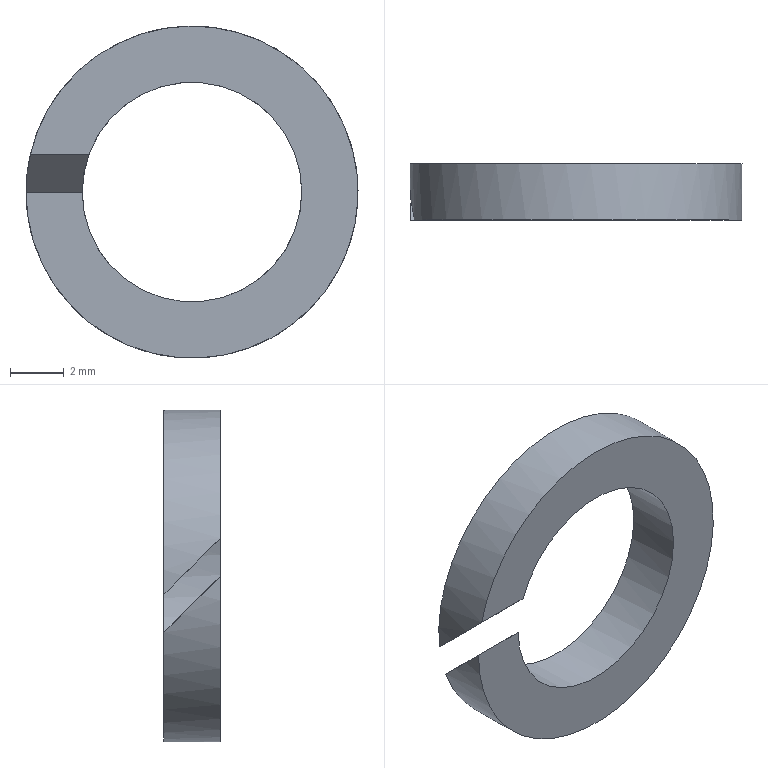Component | NX | SPRING_WASHER_8_3 | 1 solid | 6 faces | box 12.4 x 2.1 x 12.4 mm | volume 136 mm3 | plane 4 | cylinder 2 | commonest cylinder face diameters 12.4 x1 8.2 x1
STEP:
#1=CARTESIAN_POINT('',(0.,0.,0.));
#2=DIRECTION('',(0.,0.,1.));
#3=DIRECTION('',(1.,0.,0.));
#4=AXIS2_PLACEMENT_3D('',#1,#2,#3);
#5=CARTESIAN_POINT('',(-5.834,-94.,-137.1));
#6=VERTEX_POINT('',#5);
#7=CARTESIAN_POINT('',(-6.162,-94.,-135.686));
#8=VERTEX_POINT('',#7);
#9=CARTESIAN_POINT('',(-0.,-94.,-135.));
#10=DIRECTION('',(0.,-1.,0.));
#11=DIRECTION('',(-1.,0.,0.));
#12=AXIS2_PLACEMENT_3D('',#9,#10,#11);
#13=CIRCLE('',#12,6.2);
#14=CARTESIAN_POINT('',(-0.,-94.,-135.));
#15=DIRECTION('',(0.,-1.,0.));
#16=DIRECTION('',(-1.,0.,0.));
#17=AXIS2_PLACEMENT_3D('',#14,#15,#16);
#18=CYLINDRICAL_SURFACE('',#17,6.2);
#19=CARTESIAN_POINT('',(-0.,0.));
#20=DIRECTION('',(1.,0.));
#21=VECTOR('',#20,1.);
#22=LINE('',#19,#21);
#23=(GEOMETRIC_REPRESENTATION_CONTEXT(2)PARAMETRIC_REPRESENTATION_CONTEXT()REPRESENTATION_CONTEXT('',''));
#24=DEFINITIONAL_REPRESENTATION('',(#22),#23);
#25=PCURVE('',#18,#24);
#26=CARTESIAN_POINT('',(-0.,-94.,-135.));
#27=DIRECTION('',(0.,-1.,0.));
#28=DIRECTION('',(-1.,0.,0.));
#29=AXIS2_PLACEMENT_3D('',#26,#27,#28);
#30=PLANE('',#29);
#31=CARTESIAN_POINT('',(0.,0.));
#32=DIRECTION('',(1.,0.));
#33=AXIS2_PLACEMENT_2D('',#31,#32);
#34=CIRCLE('',#33,6.2);
#35=(GEOMETRIC_REPRESENTATION_CONTEXT(2)PARAMETRIC_REPRESENTATION_CONTEXT()REPRESENTATION_CONTEXT('',''));
#36=DEFINITIONAL_REPRESENTATION('',(#34),#35);
#37=PCURVE('',#30,#36);
#38=SURFACE_CURVE('',#13,(#25,#37),.PCURVE_S1.);
#39=EDGE_CURVE('',#6,#8,#38,.T.);
#40=ORIENTED_EDGE('',*,*,#39,.T.);
#41=CARTESIAN_POINT('',(-6.037,-96.1,-133.586));
#42=VERTEX_POINT('',#41);
#43=CARTESIAN_POINT('',(-0.,-94.686,-135.));
#44=DIRECTION('',(0.,0.7071,0.7071));
#45=DIRECTION('',(0.,-0.7071,0.7071));
#46=AXIS2_PLACEMENT_3D('',#43,#44,#45);
#47=ELLIPSE('',#46,8.768,6.2);
#48=CARTESIAN_POINT('',(6.394,-0.));
#49=CARTESIAN_POINT('',(6.053,2.1));
#50=B_SPLINE_CURVE_WITH_KNOTS('',1,(#48,#49),.UNSPECIFIED.,.F.,.F.,(2,2),(4.602,4.943),.PIECEWISE_BEZIER_KNOTS.);
#51=(GEOMETRIC_REPRESENTATION_CONTEXT(2)PARAMETRIC_REPRESENTATION_CONTEXT()REPRESENTATION_CONTEXT('',''));
#52=DEFINITIONAL_REPRESENTATION('',(#50),#51);
#53=PCURVE('',#18,#52);
#54=CARTESIAN_POINT('',(-9.3,-96.528,-133.158));
#55=DIRECTION('',(0.,-0.7071,-0.7071));
#56=DIRECTION('',(0.,-0.7071,0.7071));
#57=AXIS2_PLACEMENT_3D('',#54,#55,#56);
#58=PLANE('',#57);
#59=CARTESIAN_POINT('',(6.164,-9.3));
#60=CARTESIAN_POINT('',(6.164,-20.039));
#61=CARTESIAN_POINT('',(-6.989,-14.669));
#62=CARTESIAN_POINT('',(-20.141,-9.3));
#63=CARTESIAN_POINT('',(-6.989,-3.931));
#64=CARTESIAN_POINT('',(6.164,1.439));
#65=CARTESIAN_POINT('',(6.164,-9.3));
#66=(BOUNDED_CURVE()B_SPLINE_CURVE(2,(#59,#60,#61,#62,#63,#64,#65),.UNSPECIFIED.,.T.,.F.)B_SPLINE_CURVE_WITH_KNOTS((1,2,2,2,2,1),(-2.094,0.,2.094,4.189,6.283,8.378),.UNSPECIFIED.)CURVE()GEOMETRIC_REPRESENTATION_ITEM()RATIONAL_B_SPLINE_CURVE((1.,0.5,1.,0.5,1.,0.5,1.))REPRESENTATION_ITEM(''));
#67=(GEOMETRIC_REPRESENTATION_CONTEXT(2)PARAMETRIC_REPRESENTATION_CONTEXT()REPRESENTATION_CONTEXT('',''));
#68=DEFINITIONAL_REPRESENTATION('',(#66),#67);
#69=PCURVE('',#58,#68);
#70=SURFACE_CURVE('',#47,(#53,#69),.PCURVE_S1.);
#71=EDGE_CURVE('',#8,#42,#70,.T.);
#72=ORIENTED_EDGE('',*,*,#71,.T.);
#73=CARTESIAN_POINT('',(-6.2,-96.1,-135.));
#74=VERTEX_POINT('',#73);
#75=CARTESIAN_POINT('',(-0.,-96.1,-135.));
#76=DIRECTION('',(0.,-1.,0.));
#77=DIRECTION('',(-1.,0.,0.));
#78=AXIS2_PLACEMENT_3D('',#75,#76,#77);
#79=CIRCLE('',#78,6.2);
#80=CARTESIAN_POINT('',(0.,2.1));
#81=DIRECTION('',(1.,0.));
#82=VECTOR('',#81,1.);
#83=LINE('',#80,#82);
#84=(GEOMETRIC_REPRESENTATION_CONTEXT(2)PARAMETRIC_REPRESENTATION_CONTEXT()REPRESENTATION_CONTEXT('',''));
#85=DEFINITIONAL_REPRESENTATION('',(#83),#84);
#86=PCURVE('',#18,#85);
#87=CARTESIAN_POINT('',(-0.,-96.1,-135.));
#88=DIRECTION('',(0.,-1.,0.));
#89=DIRECTION('',(-1.,0.,0.));
#90=AXIS2_PLACEMENT_3D('',#87,#88,#89);
#91=PLANE('',#90);
#92=CARTESIAN_POINT('',(0.,0.));
#93=DIRECTION('',(1.,0.));
#94=AXIS2_PLACEMENT_2D('',#92,#93);
#95=CIRCLE('',#94,6.2);
#96=(GEOMETRIC_REPRESENTATION_CONTEXT(2)PARAMETRIC_REPRESENTATION_CONTEXT()REPRESENTATION_CONTEXT('',''));
#97=DEFINITIONAL_REPRESENTATION('',(#95),#96);
#98=PCURVE('',#91,#97);
#99=SURFACE_CURVE('',#79,(#86,#98),.PCURVE_S1.);
#100=EDGE_CURVE('',#74,#42,#99,.T.);
#101=ORIENTED_EDGE('',*,*,#100,.F.);
#102=CARTESIAN_POINT('',(-0.,-96.1,-135.));
#103=DIRECTION('',(0.,-0.7071,-0.7071));
#104=DIRECTION('',(0.,-0.7071,0.7071));
#105=AXIS2_PLACEMENT_3D('',#102,#103,#104);
#106=ELLIPSE('',#105,8.768,6.2);
#107=CARTESIAN_POINT('',(0.,2.1));
#108=CARTESIAN_POINT('',(0.3455,0.));
#109=B_SPLINE_CURVE_WITH_KNOTS('',1,(#107,#108),.UNSPECIFIED.,.F.,.F.,(2,2),(1.571,1.916),.PIECEWISE_BEZIER_KNOTS.);
#110=(GEOMETRIC_REPRESENTATION_CONTEXT(2)PARAMETRIC_REPRESENTATION_CONTEXT()REPRESENTATION_CONTEXT('',''));
#111=DEFINITIONAL_REPRESENTATION('',(#109),#110);
#112=PCURVE('',#18,#111);
#113=CARTESIAN_POINT('',(-9.3,-93.317,-137.783));
#114=DIRECTION('',(0.,0.7071,0.7071));
#115=DIRECTION('',(0.,0.7071,-0.7071));
#116=AXIS2_PLACEMENT_3D('',#113,#114,#115);
#117=PLANE('',#116);
#118=CARTESIAN_POINT('',(-12.704,-9.3));
#119=CARTESIAN_POINT('',(-12.704,1.439));
#120=CARTESIAN_POINT('',(0.4481,-3.931));
#121=CARTESIAN_POINT('',(13.6,-9.3));
#122=CARTESIAN_POINT('',(0.4481,-14.669));
#123=CARTESIAN_POINT('',(-12.704,-20.039));
#124=CARTESIAN_POINT('',(-12.704,-9.3));
#125=(BOUNDED_CURVE()B_SPLINE_CURVE(2,(#118,#119,#120,#121,#122,#123,#124),.UNSPECIFIED.,.T.,.F.)B_SPLINE_CURVE_WITH_KNOTS((1,2,2,2,2,1),(-2.094,0.,2.094,4.189,6.283,8.378),.UNSPECIFIED.)CURVE()GEOMETRIC_REPRESENTATION_ITEM()RATIONAL_B_SPLINE_CURVE((1.,0.5,1.,0.5,1.,0.5,1.))REPRESENTATION_ITEM(''));
#126=(GEOMETRIC_REPRESENTATION_CONTEXT(2)PARAMETRIC_REPRESENTATION_CONTEXT()REPRESENTATION_CONTEXT('',''));
#127=DEFINITIONAL_REPRESENTATION('',(#125),#126);
#128=PCURVE('',#117,#127);
#129=SURFACE_CURVE('',#106,(#112,#128),.PCURVE_S1.);
#130=EDGE_CURVE('',#74,#6,#129,.T.);
#131=ORIENTED_EDGE('',*,*,#130,.T.);
#132=EDGE_LOOP('',(#40,#72,#101,#131));
#133=FACE_BOUND('',#132,.T.);
#134=ADVANCED_FACE('',(#133),#18,.T.);
#135=CARTESIAN_POINT('',(-4.1,-96.1,-135.));
#136=VERTEX_POINT('',#135);
#137=CARTESIAN_POINT('',(-3.848,-96.1,-133.586));
#138=VERTEX_POINT('',#137);
#139=CARTESIAN_POINT('',(-0.,-96.1,-135.));
#140=DIRECTION('',(0.,-1.,0.));
#141=DIRECTION('',(-1.,0.,0.));
#142=AXIS2_PLACEMENT_3D('',#139,#140,#141);
#143=CIRCLE('',#142,4.1);
#144=CARTESIAN_POINT('',(-0.,-94.,-135.));
#145=DIRECTION('',(0.,-1.,0.));
#146=DIRECTION('',(-1.,0.,0.));
#147=AXIS2_PLACEMENT_3D('',#144,#145,#146);
#148=CYLINDRICAL_SURFACE('',#147,4.1);
#149=CARTESIAN_POINT('',(0.,2.1));
#150=DIRECTION('',(1.,0.));
#151=VECTOR('',#150,1.);
#152=LINE('',#149,#151);
#153=(GEOMETRIC_REPRESENTATION_CONTEXT(2)PARAMETRIC_REPRESENTATION_CONTEXT()REPRESENTATION_CONTEXT('',''));
#154=DEFINITIONAL_REPRESENTATION('',(#152),#153);
#155=PCURVE('',#148,#154);
#156=CARTESIAN_POINT('',(0.,0.));
#157=DIRECTION('',(1.,0.));
#158=AXIS2_PLACEMENT_2D('',#156,#157);
#159=CIRCLE('',#158,4.1);
#160=(GEOMETRIC_REPRESENTATION_CONTEXT(2)PARAMETRIC_REPRESENTATION_CONTEXT()REPRESENTATION_CONTEXT('',''));
#161=DEFINITIONAL_REPRESENTATION('',(#159),#160);
#162=PCURVE('',#91,#161);
#163=SURFACE_CURVE('',#143,(#155,#162),.PCURVE_S1.);
#164=EDGE_CURVE('',#136,#138,#163,.T.);
#165=ORIENTED_EDGE('',*,*,#164,.F.);
#166=CARTESIAN_POINT('',(-3.521,-94.,-137.1));
#167=VERTEX_POINT('',#166);
#168=CARTESIAN_POINT('',(-0.,-96.1,-135.));
#169=DIRECTION('',(0.,-0.7071,-0.7071));
#170=DIRECTION('',(0.,-0.7071,0.7071));
#171=AXIS2_PLACEMENT_3D('',#168,#169,#170);
#172=ELLIPSE('',#171,5.798,4.1);
#173=CARTESIAN_POINT('',(0.,2.1));
#174=CARTESIAN_POINT('',(0.5377,0.));
#175=B_SPLINE_CURVE_WITH_KNOTS('',1,(#173,#174),.UNSPECIFIED.,.F.,.F.,(2,2),(1.571,2.109),.PIECEWISE_BEZIER_KNOTS.);
#176=(GEOMETRIC_REPRESENTATION_CONTEXT(2)PARAMETRIC_REPRESENTATION_CONTEXT()REPRESENTATION_CONTEXT('',''));
#177=DEFINITIONAL_REPRESENTATION('',(#175),#176);
#178=PCURVE('',#148,#177);
#179=CARTESIAN_POINT('',(-9.734,-9.3));
#180=CARTESIAN_POINT('',(-9.734,-2.199));
#181=CARTESIAN_POINT('',(-1.037,-5.749));
#182=CARTESIAN_POINT('',(7.661,-9.3));
#183=CARTESIAN_POINT('',(-1.037,-12.851));
#184=CARTESIAN_POINT('',(-9.734,-16.401));
#185=CARTESIAN_POINT('',(-9.734,-9.3));
#186=(BOUNDED_CURVE()B_SPLINE_CURVE(2,(#179,#180,#181,#182,#183,#184,#185),.UNSPECIFIED.,.T.,.F.)B_SPLINE_CURVE_WITH_KNOTS((1,2,2,2,2,1),(-2.094,0.,2.094,4.189,6.283,8.378),.UNSPECIFIED.)CURVE()GEOMETRIC_REPRESENTATION_ITEM()RATIONAL_B_SPLINE_CURVE((1.,0.5,1.,0.5,1.,0.5,1.))REPRESENTATION_ITEM(''));
#187=(GEOMETRIC_REPRESENTATION_CONTEXT(2)PARAMETRIC_REPRESENTATION_CONTEXT()REPRESENTATION_CONTEXT('',''));
#188=DEFINITIONAL_REPRESENTATION('',(#186),#187);
#189=PCURVE('',#117,#188);
#190=SURFACE_CURVE('',#172,(#178,#189),.PCURVE_S1.);
#191=EDGE_CURVE('',#136,#167,#190,.T.);
#192=ORIENTED_EDGE('',*,*,#191,.T.);
#193=CARTESIAN_POINT('',(-4.042,-94.,-135.686));
#194=VERTEX_POINT('',#193);
#195=CARTESIAN_POINT('',(-0.,-94.,-135.));
#196=DIRECTION('',(0.,-1.,0.));
#197=DIRECTION('',(-1.,0.,0.));
#198=AXIS2_PLACEMENT_3D('',#195,#196,#197);
#199=CIRCLE('',#198,4.1);
#200=CARTESIAN_POINT('',(-0.,0.));
#201=DIRECTION('',(1.,0.));
#202=VECTOR('',#201,1.);
#203=LINE('',#200,#202);
#204=(GEOMETRIC_REPRESENTATION_CONTEXT(2)PARAMETRIC_REPRESENTATION_CONTEXT()REPRESENTATION_CONTEXT('',''));
#205=DEFINITIONAL_REPRESENTATION('',(#203),#204);
#206=PCURVE('',#148,#205);
#207=CARTESIAN_POINT('',(0.,0.));
#208=DIRECTION('',(1.,0.));
#209=AXIS2_PLACEMENT_2D('',#207,#208);
#210=CIRCLE('',#209,4.1);
#211=(GEOMETRIC_REPRESENTATION_CONTEXT(2)PARAMETRIC_REPRESENTATION_CONTEXT()REPRESENTATION_CONTEXT('',''));
#212=DEFINITIONAL_REPRESENTATION('',(#210),#211);
#213=PCURVE('',#30,#212);
#214=SURFACE_CURVE('',#199,(#206,#213),.PCURVE_S1.);
#215=EDGE_CURVE('',#167,#194,#214,.T.);
#216=ORIENTED_EDGE('',*,*,#215,.T.);
#217=CARTESIAN_POINT('',(-0.,-94.686,-135.));
#218=DIRECTION('',(0.,0.7071,0.7071));
#219=DIRECTION('',(0.,-0.7071,0.7071));
#220=AXIS2_PLACEMENT_3D('',#217,#218,#219);
#221=ELLIPSE('',#220,5.798,4.1);
#222=CARTESIAN_POINT('',(6.451,-0.));
#223=CARTESIAN_POINT('',(5.931,2.1));
#224=B_SPLINE_CURVE_WITH_KNOTS('',1,(#222,#223),.UNSPECIFIED.,.F.,.F.,(2,2),(4.544,5.065),.PIECEWISE_BEZIER_KNOTS.);
#225=(GEOMETRIC_REPRESENTATION_CONTEXT(2)PARAMETRIC_REPRESENTATION_CONTEXT()REPRESENTATION_CONTEXT('',''));
#226=DEFINITIONAL_REPRESENTATION('',(#224),#225);
#227=PCURVE('',#148,#226);
#228=CARTESIAN_POINT('',(3.194,-9.3));
#229=CARTESIAN_POINT('',(3.194,-16.401));
#230=CARTESIAN_POINT('',(-5.504,-12.851));
#231=CARTESIAN_POINT('',(-14.201,-9.3));
#232=CARTESIAN_POINT('',(-5.504,-5.749));
#233=CARTESIAN_POINT('',(3.194,-2.199));
#234=CARTESIAN_POINT('',(3.194,-9.3));
#235=(BOUNDED_CURVE()B_SPLINE_CURVE(2,(#228,#229,#230,#231,#232,#233,#234),.UNSPECIFIED.,.T.,.F.)B_SPLINE_CURVE_WITH_KNOTS((1,2,2,2,2,1),(-2.094,0.,2.094,4.189,6.283,8.378),.UNSPECIFIED.)CURVE()GEOMETRIC_REPRESENTATION_ITEM()RATIONAL_B_SPLINE_CURVE((1.,0.5,1.,0.5,1.,0.5,1.))REPRESENTATION_ITEM(''));
#236=(GEOMETRIC_REPRESENTATION_CONTEXT(2)PARAMETRIC_REPRESENTATION_CONTEXT()REPRESENTATION_CONTEXT('',''));
#237=DEFINITIONAL_REPRESENTATION('',(#235),#236);
#238=PCURVE('',#58,#237);
#239=SURFACE_CURVE('',#221,(#227,#238),.PCURVE_S1.);
#240=EDGE_CURVE('',#194,#138,#239,.T.);
#241=ORIENTED_EDGE('',*,*,#240,.T.);
#242=EDGE_LOOP('',(#165,#192,#216,#241));
#243=FACE_BOUND('',#242,.F.);
#244=ADVANCED_FACE('',(#243),#148,.F.);
#245=CARTESIAN_POINT('',(-0.,-94.,-135.686));
#246=DIRECTION('',(1.,0.,0.));
#247=VECTOR('',#246,1.);
#248=LINE('',#245,#247);
#249=CARTESIAN_POINT('',(0.,0.6858));
#250=DIRECTION('',(-1.,0.));
#251=VECTOR('',#250,1.);
#252=LINE('',#249,#251);
#253=(GEOMETRIC_REPRESENTATION_CONTEXT(2)PARAMETRIC_REPRESENTATION_CONTEXT()REPRESENTATION_CONTEXT('',''));
#254=DEFINITIONAL_REPRESENTATION('',(#252),#253);
#255=PCURVE('',#30,#254);
#256=CARTESIAN_POINT('',(-3.574,-9.3));
#257=DIRECTION('',(0.,-1.));
#258=VECTOR('',#257,1.);
#259=LINE('',#256,#258);
#260=(GEOMETRIC_REPRESENTATION_CONTEXT(2)PARAMETRIC_REPRESENTATION_CONTEXT()REPRESENTATION_CONTEXT('',''));
#261=DEFINITIONAL_REPRESENTATION('',(#259),#260);
#262=PCURVE('',#58,#261);
#263=SURFACE_CURVE('',#248,(#255,#262),.PCURVE_S1.);
#264=EDGE_CURVE('',#8,#194,#263,.T.);
#265=ORIENTED_EDGE('',*,*,#264,.F.);
#266=ORIENTED_EDGE('',*,*,#39,.F.);
#267=CARTESIAN_POINT('',(-0.,-94.,-137.1));
#268=DIRECTION('',(-1.,0.,0.));
#269=VECTOR('',#268,1.);
#270=LINE('',#267,#269);
#271=CARTESIAN_POINT('',(0.,2.1));
#272=DIRECTION('',(1.,0.));
#273=VECTOR('',#272,1.);
#274=LINE('',#271,#273);
#275=(GEOMETRIC_REPRESENTATION_CONTEXT(2)PARAMETRIC_REPRESENTATION_CONTEXT()REPRESENTATION_CONTEXT('',''));
#276=DEFINITIONAL_REPRESENTATION('',(#274),#275);
#277=PCURVE('',#30,#276);
#278=CARTESIAN_POINT('',(-0.9661,-9.3));
#279=DIRECTION('',(0.,1.));
#280=VECTOR('',#279,1.);
#281=LINE('',#278,#280);
#282=(GEOMETRIC_REPRESENTATION_CONTEXT(2)PARAMETRIC_REPRESENTATION_CONTEXT()REPRESENTATION_CONTEXT('',''));
#283=DEFINITIONAL_REPRESENTATION('',(#281),#282);
#284=PCURVE('',#117,#283);
#285=SURFACE_CURVE('',#270,(#277,#284),.PCURVE_S1.);
#286=EDGE_CURVE('',#167,#6,#285,.T.);
#287=ORIENTED_EDGE('',*,*,#286,.F.);
#288=ORIENTED_EDGE('',*,*,#215,.T.);
#289=EDGE_LOOP('',(#265,#266,#287,#288));
#290=FACE_BOUND('',#289,.T.);
#291=ADVANCED_FACE('',(#290),#30,.F.);
#292=ORIENTED_EDGE('',*,*,#100,.T.);
#293=CARTESIAN_POINT('',(-0.,-96.1,-133.586));
#294=DIRECTION('',(1.,0.,0.));
#295=VECTOR('',#294,1.);
#296=LINE('',#293,#295);
#297=CARTESIAN_POINT('',(0.,-1.414));
#298=DIRECTION('',(-1.,0.));
#299=VECTOR('',#298,1.);
#300=LINE('',#297,#299);
#301=(GEOMETRIC_REPRESENTATION_CONTEXT(2)PARAMETRIC_REPRESENTATION_CONTEXT()REPRESENTATION_CONTEXT('',''));
#302=DEFINITIONAL_REPRESENTATION('',(#300),#301);
#303=PCURVE('',#91,#302);
#304=CARTESIAN_POINT('',(-0.6046,-9.3));
#305=DIRECTION('',(0.,-1.));
#306=VECTOR('',#305,1.);
#307=LINE('',#304,#306);
#308=(GEOMETRIC_REPRESENTATION_CONTEXT(2)PARAMETRIC_REPRESENTATION_CONTEXT()REPRESENTATION_CONTEXT('',''));
#309=DEFINITIONAL_REPRESENTATION('',(#307),#308);
#310=PCURVE('',#58,#309);
#311=SURFACE_CURVE('',#296,(#303,#310),.PCURVE_S1.);
#312=EDGE_CURVE('',#42,#138,#311,.T.);
#313=ORIENTED_EDGE('',*,*,#312,.T.);
#314=ORIENTED_EDGE('',*,*,#164,.F.);
#315=CARTESIAN_POINT('',(-0.,-96.1,-135.));
#316=DIRECTION('',(-1.,0.,0.));
#317=VECTOR('',#316,1.);
#318=LINE('',#315,#317);
#319=CARTESIAN_POINT('',(0.,0.));
#320=DIRECTION('',(1.,0.));
#321=VECTOR('',#320,1.);
#322=LINE('',#319,#321);
#323=(GEOMETRIC_REPRESENTATION_CONTEXT(2)PARAMETRIC_REPRESENTATION_CONTEXT()REPRESENTATION_CONTEXT('',''));
#324=DEFINITIONAL_REPRESENTATION('',(#322),#323);
#325=PCURVE('',#91,#324);
#326=CARTESIAN_POINT('',(-3.936,-9.3));
#327=DIRECTION('',(0.,1.));
#328=VECTOR('',#327,1.);
#329=LINE('',#326,#328);
#330=(GEOMETRIC_REPRESENTATION_CONTEXT(2)PARAMETRIC_REPRESENTATION_CONTEXT()REPRESENTATION_CONTEXT('',''));
#331=DEFINITIONAL_REPRESENTATION('',(#329),#330);
#332=PCURVE('',#117,#331);
#333=SURFACE_CURVE('',#318,(#325,#332),.PCURVE_S1.);
#334=EDGE_CURVE('',#136,#74,#333,.T.);
#335=ORIENTED_EDGE('',*,*,#334,.T.);
#336=EDGE_LOOP('',(#292,#313,#314,#335));
#337=FACE_BOUND('',#336,.T.);
#338=ADVANCED_FACE('',(#337),#91,.T.);
#339=ORIENTED_EDGE('',*,*,#286,.T.);
#340=ORIENTED_EDGE('',*,*,#130,.F.);
#341=ORIENTED_EDGE('',*,*,#334,.F.);
#342=ORIENTED_EDGE('',*,*,#191,.T.);
#343=EDGE_LOOP('',(#339,#340,#341,#342));
#344=FACE_BOUND('',#343,.T.);
#345=ADVANCED_FACE('',(#344),#117,.T.);
#346=ORIENTED_EDGE('',*,*,#264,.T.);
#347=ORIENTED_EDGE('',*,*,#240,.T.);
#348=ORIENTED_EDGE('',*,*,#312,.F.);
#349=ORIENTED_EDGE('',*,*,#71,.F.);
#350=EDGE_LOOP('',(#346,#347,#348,#349));
#351=FACE_BOUND('',#350,.T.);
#352=ADVANCED_FACE('',(#351),#58,.T.);
#353=CLOSED_SHELL('',(#134,#244,#291,#338,#345,#352));
#354=MANIFOLD_SOLID_BREP('',#353);
#355=(LENGTH_UNIT()NAMED_UNIT(*)SI_UNIT(.MILLI.,.METRE.));
#356=UNCERTAINTY_MEASURE_WITH_UNIT(LENGTH_MEASURE(0.02),#355,'','');
#357=(NAMED_UNIT(*)PLANE_ANGLE_UNIT()SI_UNIT($,.RADIAN.));
#358=(NAMED_UNIT(*)SI_UNIT($,.STERADIAN.)SOLID_ANGLE_UNIT());
#359=(GEOMETRIC_REPRESENTATION_CONTEXT(3)GLOBAL_UNCERTAINTY_ASSIGNED_CONTEXT((#356))GLOBAL_UNIT_ASSIGNED_CONTEXT((#355,#357,#358))REPRESENTATION_CONTEXT('',''));
#360=ADVANCED_BREP_SHAPE_REPRESENTATION('',(#4,#354),#359);